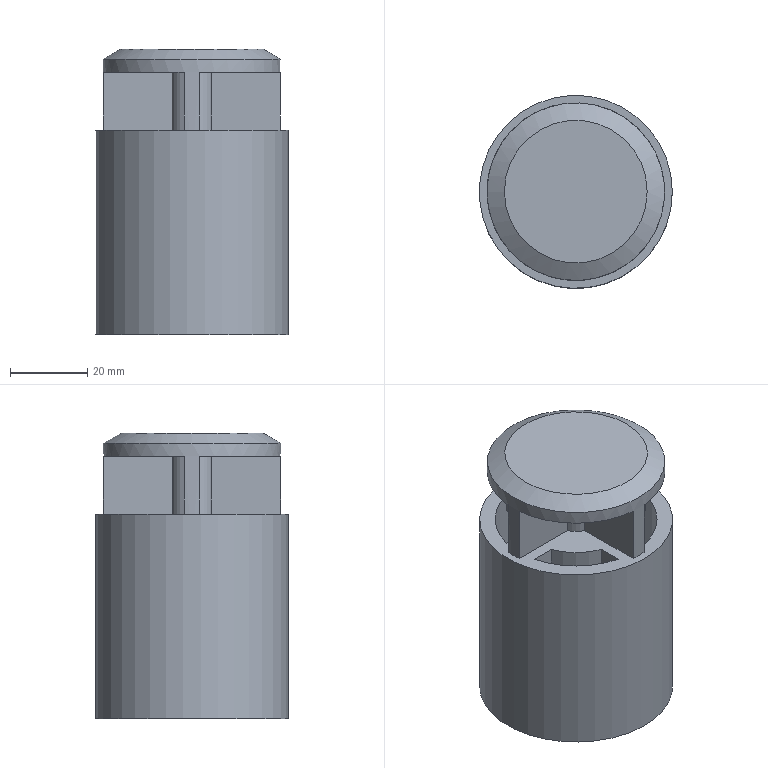Component | NX | VALVE_DISC | 1 solid | 145 faces | volume 62411 mm3 | plane 93 | cylinder 39 | spline 12 | cone 1 | commonest cylinder face diameters 42 x8 30 x8 4.134 x4 15 x4 11 x4 5 x4 19.8 x4 46 x1